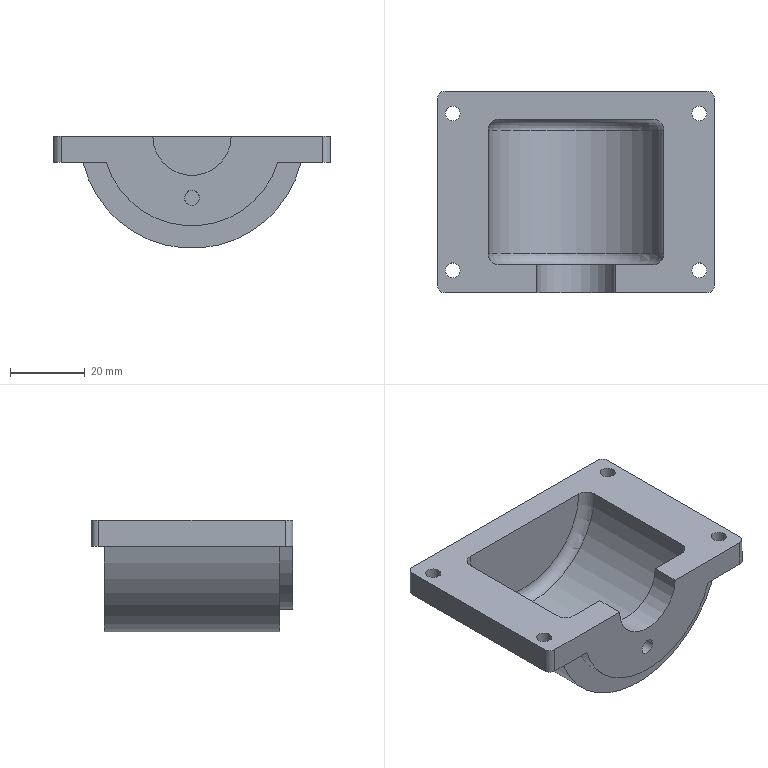Component | NX | BOTTOM_CASING | 1 solid | 25 faces | volume 41542 mm3 | cylinder 13 | plane 10 | torus 2 | commonest cylinder face diameters 4 x9 60 x1 48 x1 47 x1 21 x1